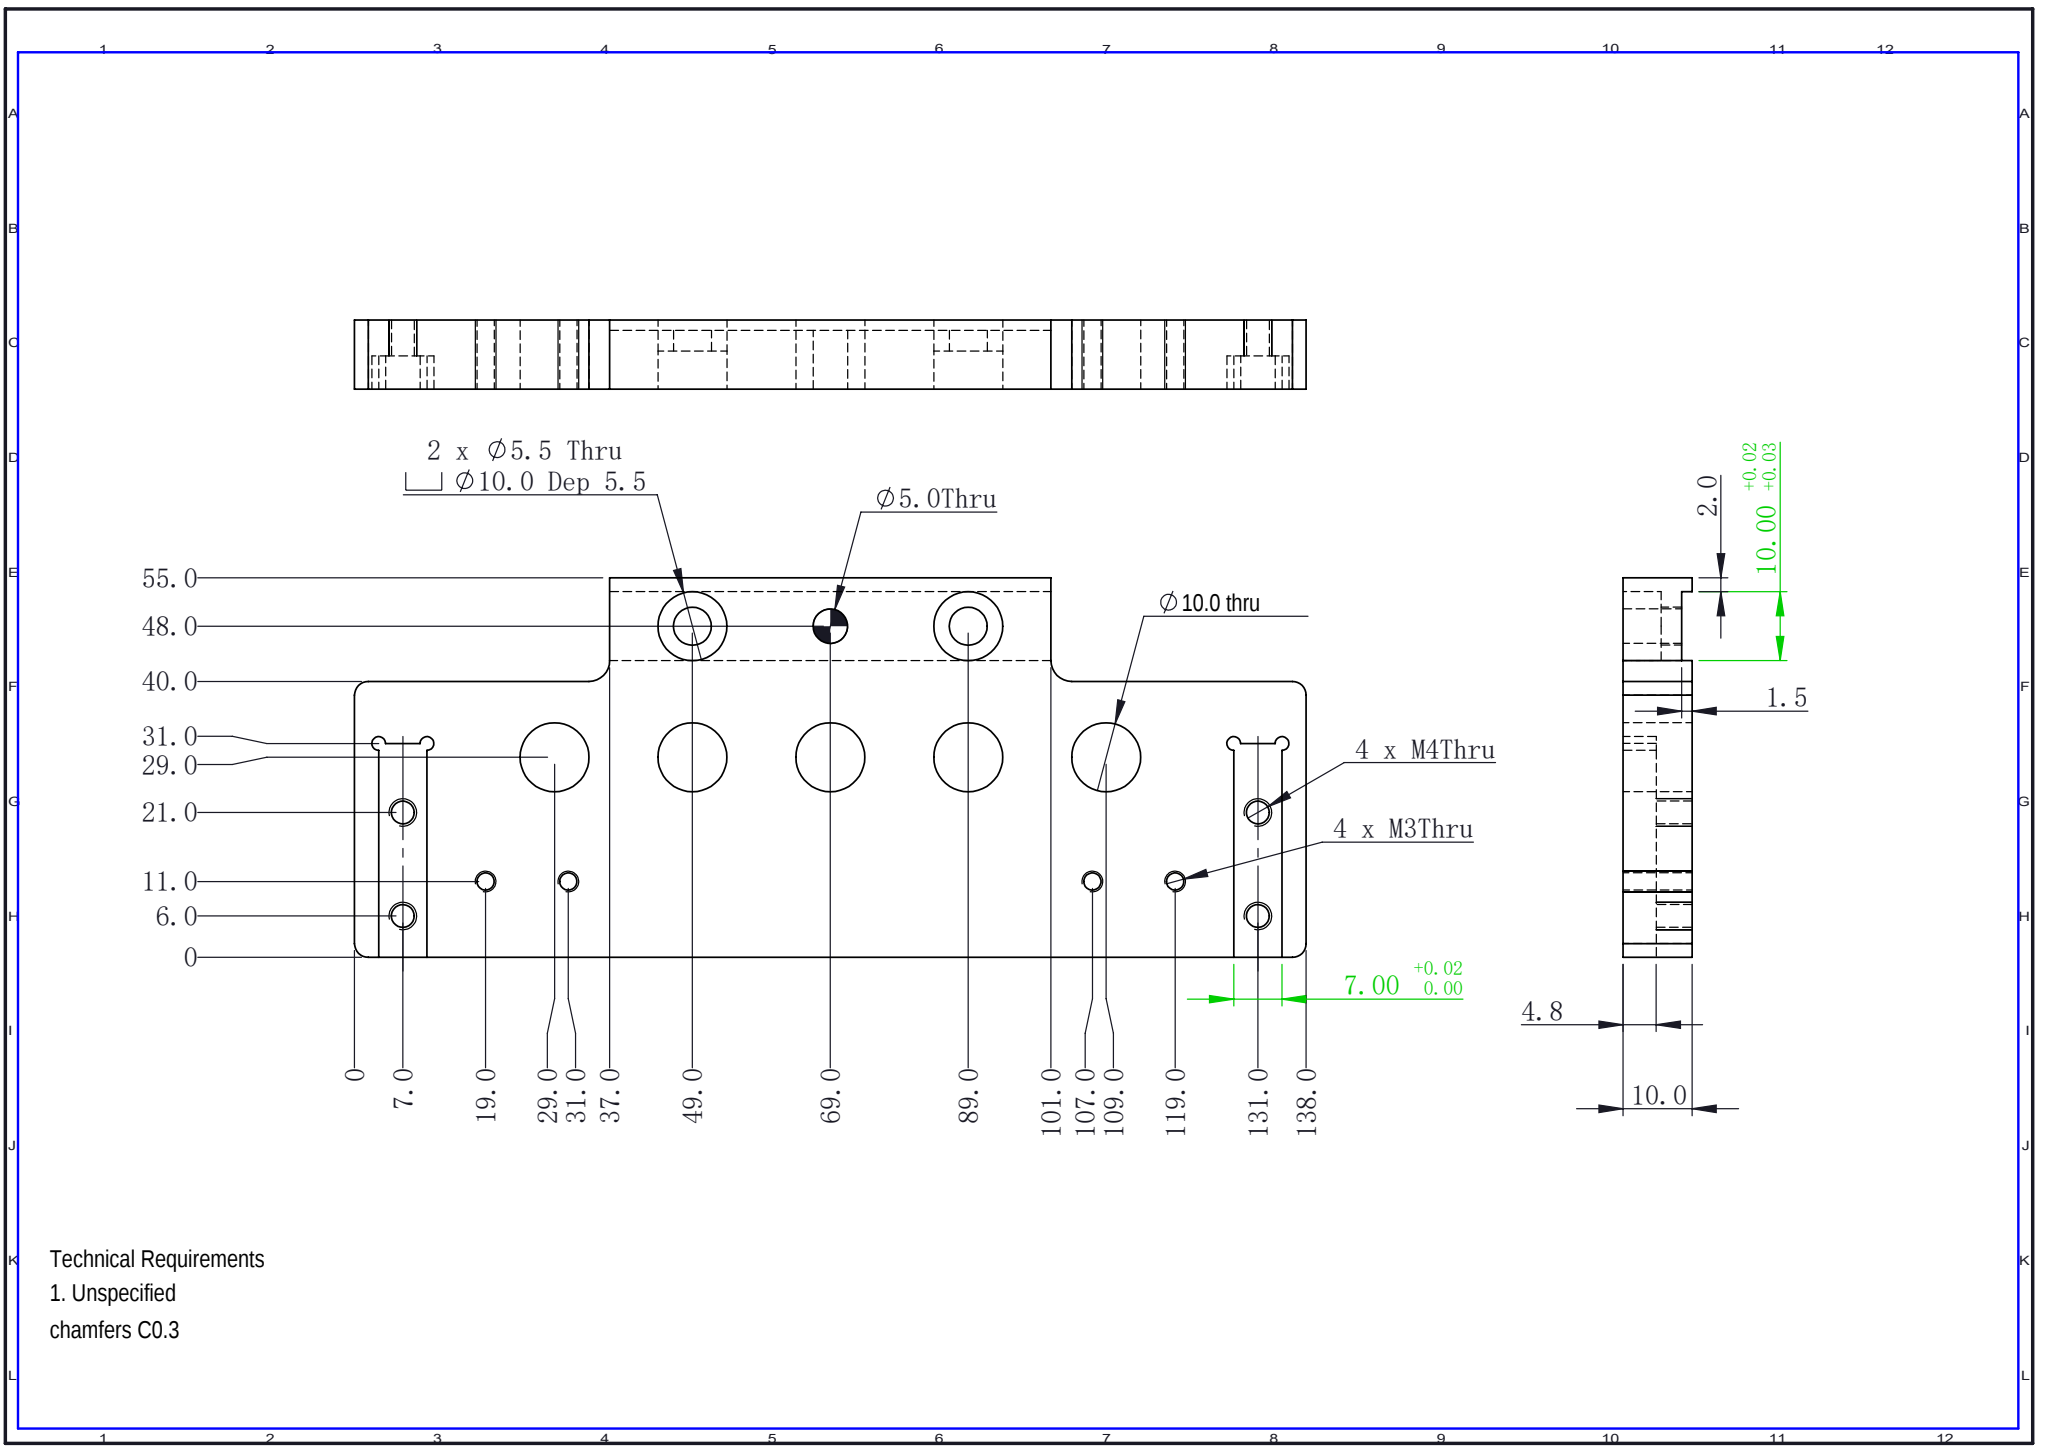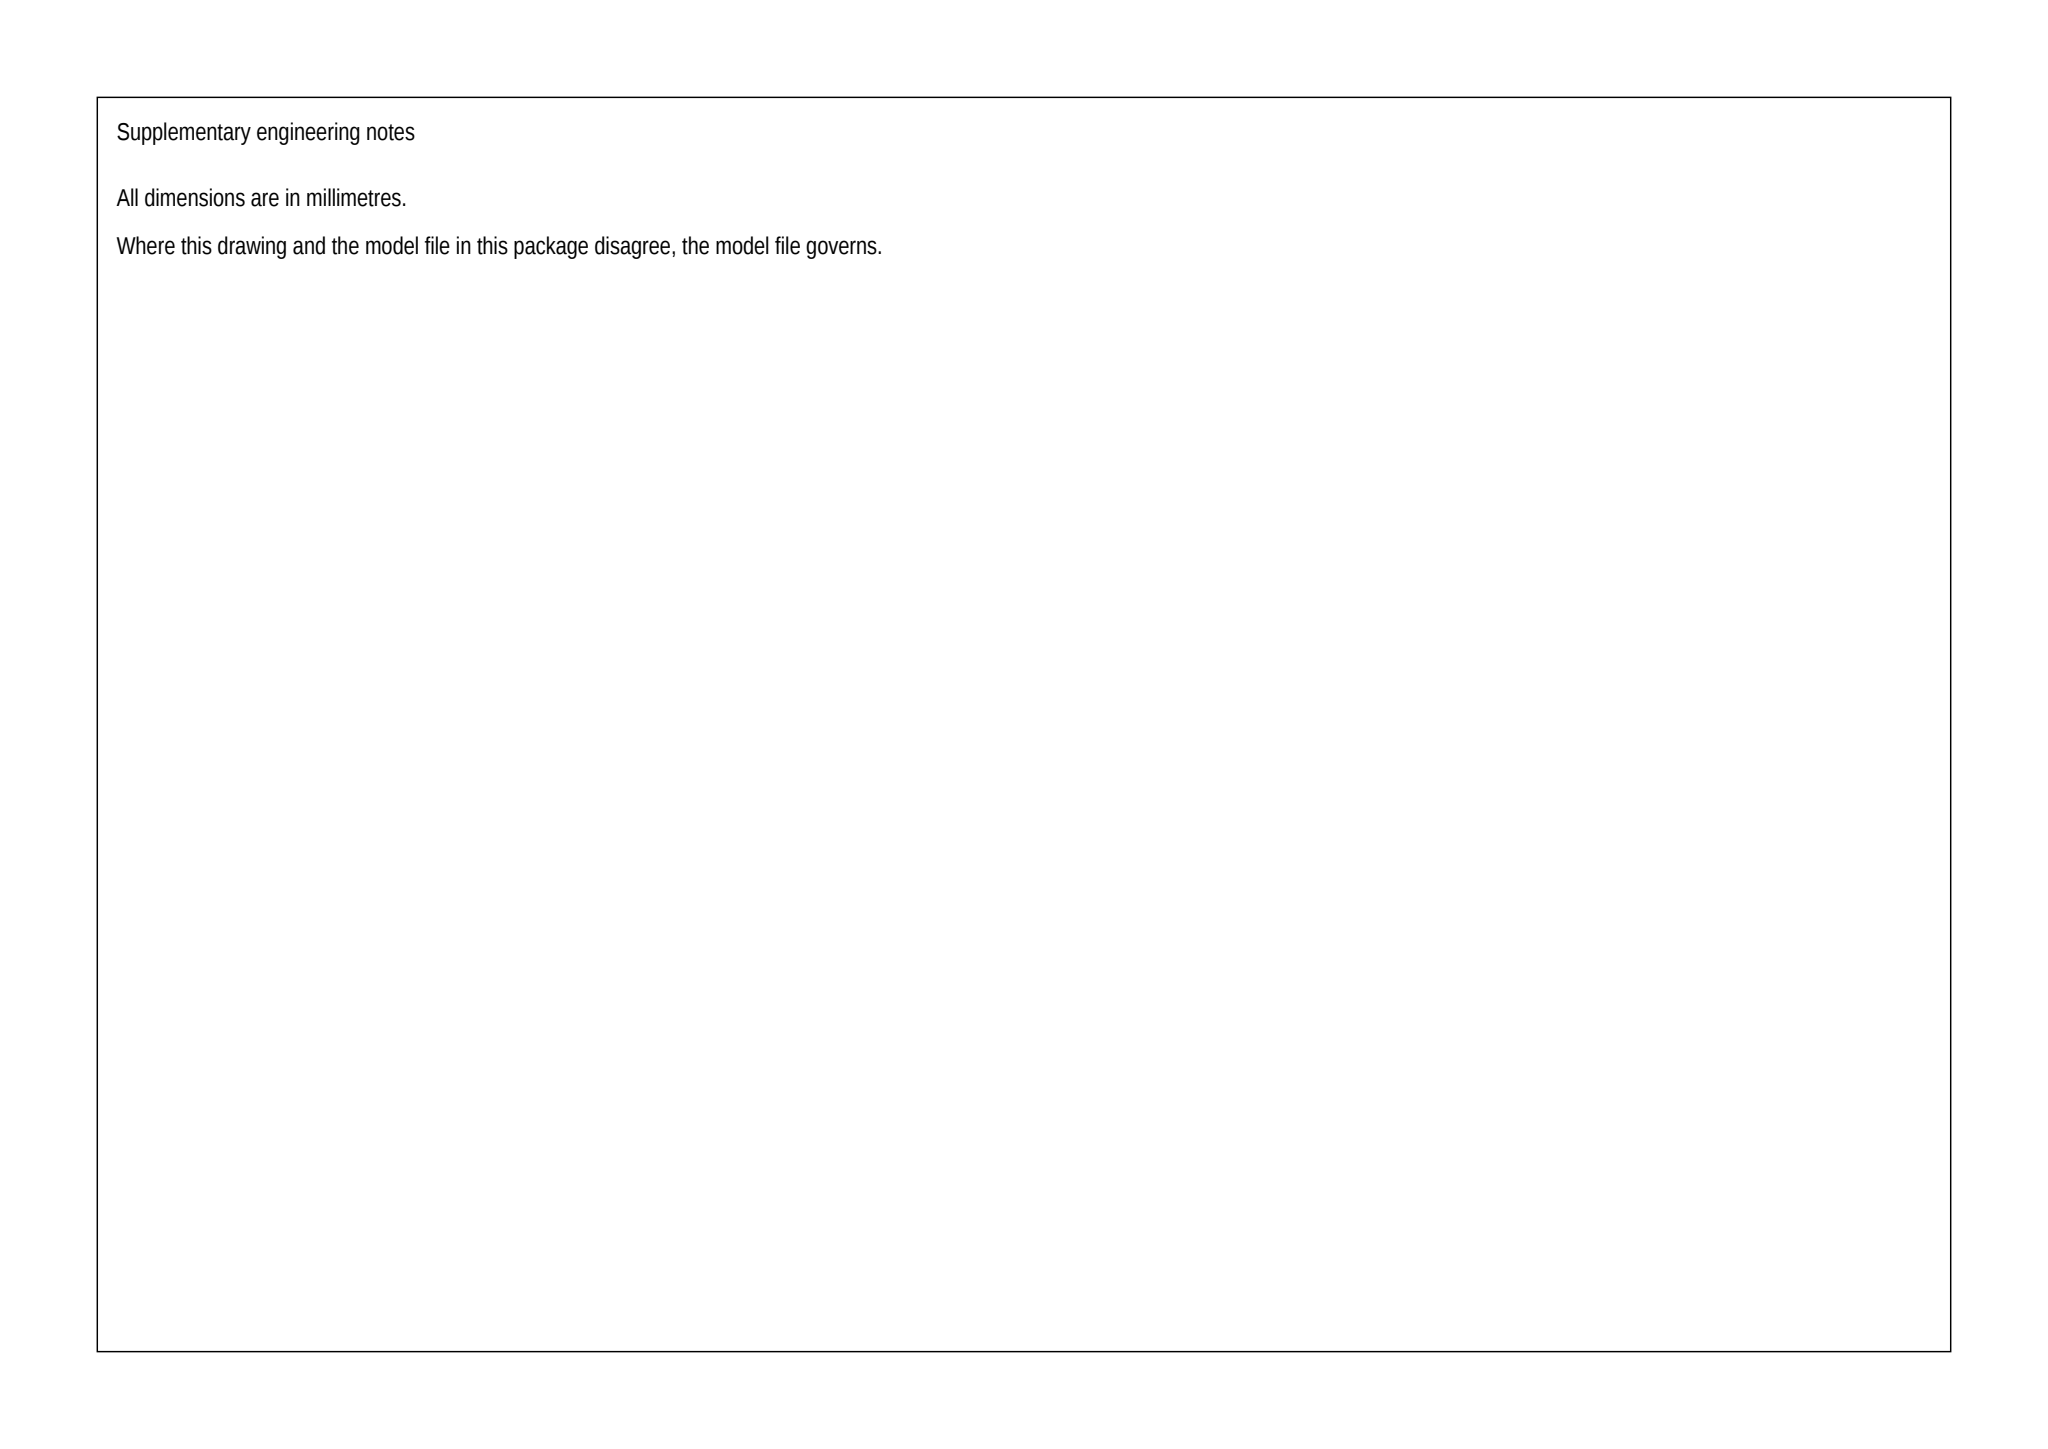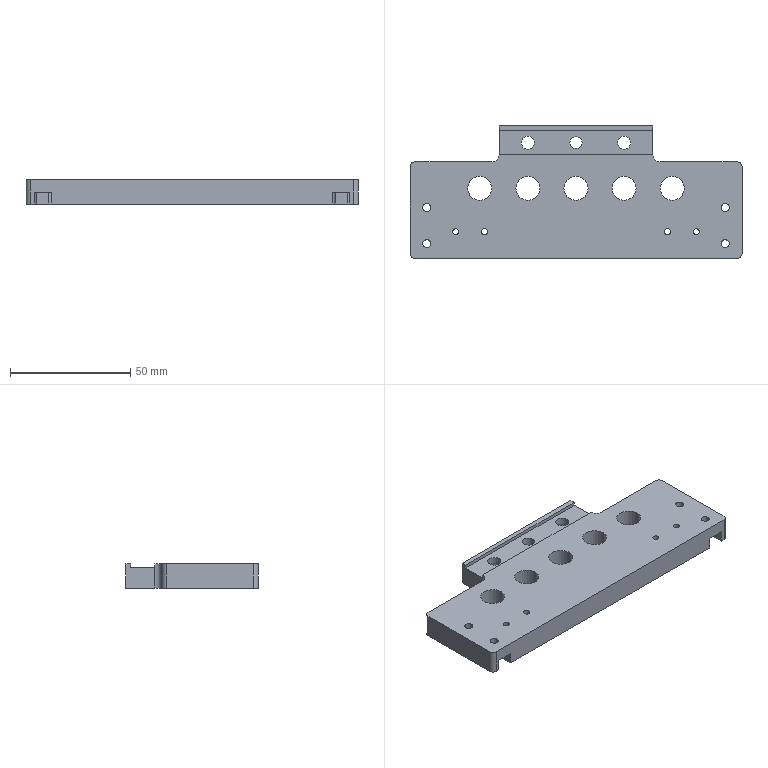Part | SolidWorks | mm | 1 solid | 72 faces | box 138 x 55 x 10 mm | volume 56241 mm3 | cylinder 48 | plane 24 | commonest cylinder face diameters 10 x14 2.5 x8 3.3 x8 2 x6 5.5 x4 4 x4 5 x2 6 x2
Drawing notes:
4 x R2 CORNER RAD FULL HT AT X=2 & 136, Y=2 & 38 | from the solid: Ø4.0 z-cyls L=10.0 at (2,2),(2,38),(136,2),(136,38)
2 x R3 INT FILLET AT TAB STEP, X=34 & 104, Y=43 | from the solid: Ø6.0 z-cyls L=10.0 at (34,43) and (104,43)
2 x SLOT 7.00W R1 ENDS DP4.8 FROM BTM, Y0-31, X3.5/10.5 & 127.5/134.5 | from the solid: x-planes 3.5/10.5 & 127.5/134.5; Ø2.0 end cyls at y=31 L=4.8; z-plane 4.8
4 x M4 THRU, NO CBORE, OPEN INTO 7.00 SLOT, THD LG 5.2 | from the solid: Ø3.3 at (7,6),(7,21),(131,6),(131,21) L=5.2 = 10.0-4.8 slot floor
TAB RECESS 1.5 DP (8.5 THK) X=37-101, Y=43-53, 10.00 W, 2.0 FROM Y=55 | from the solid: z-plane 8.5; x-planes 37/101; y-planes 43/53 (10.00), 55-53=2.0
5 x Ø10.0 THRU AT Y=29.0 (X=29,49,69,89,109) | from the solid: cylinders dia 10.0, axis z, len 10.0 at (29,29),(49,29),(69,29),(89,29),(109,29); part thk 10.0
build123d program:
from build123d import *

# Parameters (mm, degrees)
SKETCH1_W                                       = 138
SKETCH1_H                                       = 90
BOSS_EXTRUDE1_DEPTH                             = 10
SKETCH2_W                                       = 64
SKETCH2_H                                       = 15
BOSS_EXTRUDE2_DEPTH                             = 10
FILLET1_R                                       = 3
FILLET2_R                                       = 2
SKETCH6_R                                       = 5
CUT_EXTRUDE3_DEPTH                              = 92.984
SKETCH8_W                                       = 64
SKETCH8_H                                       = 10
CUT_EXTRUDE4_DEPTH                              = 1.5
SIZE_MM_DOWEL_PIN_HOLE1_D                       = 5
M5_HEX_SOCKET_HEAD_CAP_SCREW_CBORE1_D           = 5.5
M5_HEX_SOCKET_HEAD_CAP_SCREW_CBORE1_CBORE_D     = 10
M5_HEX_SOCKET_HEAD_CAP_SCREW_CBORE1_CBORE_DEPTH = 5.5
SKETCH13_W                                      = 138
SKETCH13_H                                      = 50
CUT_EXTRUDE5_DEPTH                              = 92.984
FILLET3_R                                       = 2
SKETCH14_W                                      = 7
SKETCH14_H                                      = 31
CUT_EXTRUDE6_DEPTH                              = 4.8
SKETCH15_R                                      = 1
CUT_EXTRUDE7_DEPTH                              = 4.8
M4_TAPPED_HOLE1_D                               = 3.3
M3_TAPPED_HOLE1_D                               = 2.5


with BuildPart() as part:
    # Sketch1 → Boss-Extrude1 (new body)
    with BuildSketch(Plane.XY):
        Rectangle(SKETCH1_W, SKETCH1_H)
    extrude(amount=BOSS_EXTRUDE1_DEPTH)

    # Sketch2 → Boss-Extrude2 (add)
    with BuildSketch(Plane.XY.offset(10)):
        with Locations((0, 52.5)):
            Rectangle(SKETCH2_W, SKETCH2_H)
    extrude(amount=-BOSS_EXTRUDE2_DEPTH)

    # Fillet1
    fillet1_edges = [part.edges().sort_by_distance(p)[0] for p in [
        (-32, 45, 5),
        (32, 45, 5),
    ]]
    fillet(fillet1_edges, radius=FILLET1_R)

    # Fillet2
    fillet2_edges = [part.edges().sort_by_distance(p)[0] for p in [
        (69, -45, 5),
        (-69, -45, 5),
        (-69, 45, 5),
        (69, 45, 5),
    ]]
    fillet(fillet2_edges, radius=FILLET2_R)

    # Sketch6 → Cut-Extrude3 (cut, through all)
    with BuildSketch(Plane.XY.offset(10)):
        with Locations((0, -6.5)):
            Circle(SKETCH6_R)
        with Locations((0, 34)):
            Circle(SKETCH6_R)
        with Locations((20, -6.5)):
            Circle(SKETCH6_R)
        with Locations((20, 34)):
            Circle(SKETCH6_R)
        with Locations((40, -6.5)):
            Circle(SKETCH6_R)
        with Locations((40, 34)):
            Circle(SKETCH6_R)
        with Locations((-20, 34)):
            Circle(SKETCH6_R)
        with Locations((-40, 34)):
            Circle(SKETCH6_R)
        with Locations((-40, -6.5)):
            Circle(SKETCH6_R)
        with Locations((-20, -6.5)):
            Circle(SKETCH6_R)
        with Locations((40, -31)):
            Circle(SKETCH6_R)
        with Locations((20, -34.5)):
            Circle(SKETCH6_R)
        with Locations((0, -31)):
            Circle(SKETCH6_R)
        with Locations((-20, -34.5)):
            Circle(SKETCH6_R)
        with Locations((-40, -31)):
            Circle(SKETCH6_R)
    extrude(amount=-CUT_EXTRUDE3_DEPTH, mode=Mode.SUBTRACT)

    # Sketch8 → Cut-Extrude4 (cut)
    with BuildSketch(Plane.XY.offset(10)):
        with Locations((0, 53)):
            Rectangle(SKETCH8_W, SKETCH8_H)
    extrude(amount=-CUT_EXTRUDE4_DEPTH, mode=Mode.SUBTRACT)

    # Size mm Dowel Pin Hole1 (through all)
    with Locations(Plane.XY.offset(8.5)):
        with Locations((0, 53)):
            Hole(SIZE_MM_DOWEL_PIN_HOLE1_D / 2)

    # M5 Hex Socket Head Cap Screw CBORE1 (through all)
    with Locations(Plane(origin=(0, 0, 0), x_dir=(-1, 0, 0), z_dir=(0, 0, -1))):
        with Locations((20, 53), (-20, 53)):
            CounterBoreHole(M5_HEX_SOCKET_HEAD_CAP_SCREW_CBORE1_D / 2, M5_HEX_SOCKET_HEAD_CAP_SCREW_CBORE1_CBORE_D / 2, M5_HEX_SOCKET_HEAD_CAP_SCREW_CBORE1_CBORE_DEPTH)

    # Sketch13 → Cut-Extrude5 (cut, through all)
    with BuildSketch(Plane(origin=(0, 0, 0), x_dir=(-1, 0, 0), z_dir=(0, 0, -1))):
        with Locations((0, -20)):
            Rectangle(SKETCH13_W, SKETCH13_H)
    extrude(amount=-CUT_EXTRUDE5_DEPTH, mode=Mode.SUBTRACT)

    # Fillet3
    fillet3_edges = [part.edges().sort_by_distance(p)[0] for p in [
        (-69, 5, 5),
        (69, 5, 5),
    ]]
    fillet(fillet3_edges, radius=FILLET3_R)

    # Sketch14 → Cut-Extrude6 (cut)
    with BuildSketch(Plane.XY):
        with Locations((-62, 20.5)):
            Rectangle(SKETCH14_W, SKETCH14_H)
        with Locations((62, 20.5)):
            Rectangle(SKETCH14_W, SKETCH14_H)
    extrude(amount=CUT_EXTRUDE6_DEPTH, mode=Mode.SUBTRACT)

    # Sketch15 → Cut-Extrude7 (cut)
    with BuildSketch(Plane.XY):
        with Locations((-58.5, 36)):
            Circle(SKETCH15_R)
        with Locations((-65.5, 36)):
            Circle(SKETCH15_R)
        with Locations((65.5, 36)):
            Circle(SKETCH15_R)
        with Locations((58.5, 36)):
            Circle(SKETCH15_R)
    extrude(amount=CUT_EXTRUDE7_DEPTH, mode=Mode.SUBTRACT)

    # M4 Tapped Hole1 (through all)
    with Locations(Plane(origin=(0, 0, 4.8), x_dir=(-1, 0, 0), z_dir=(0, 0, -1))):
        with Locations((-62, 11), (-62, 26), (62, 11), (62, 26)):
            Hole(M4_TAPPED_HOLE1_D / 2)

    # M3 Tapped Hole1 (through all)
    with Locations(Plane.XY.offset(10)):
        with Locations((-50, 16), (-38, 16), (38, 16), (50, 16)):
            Hole(M3_TAPPED_HOLE1_D / 2)


solid = part.part